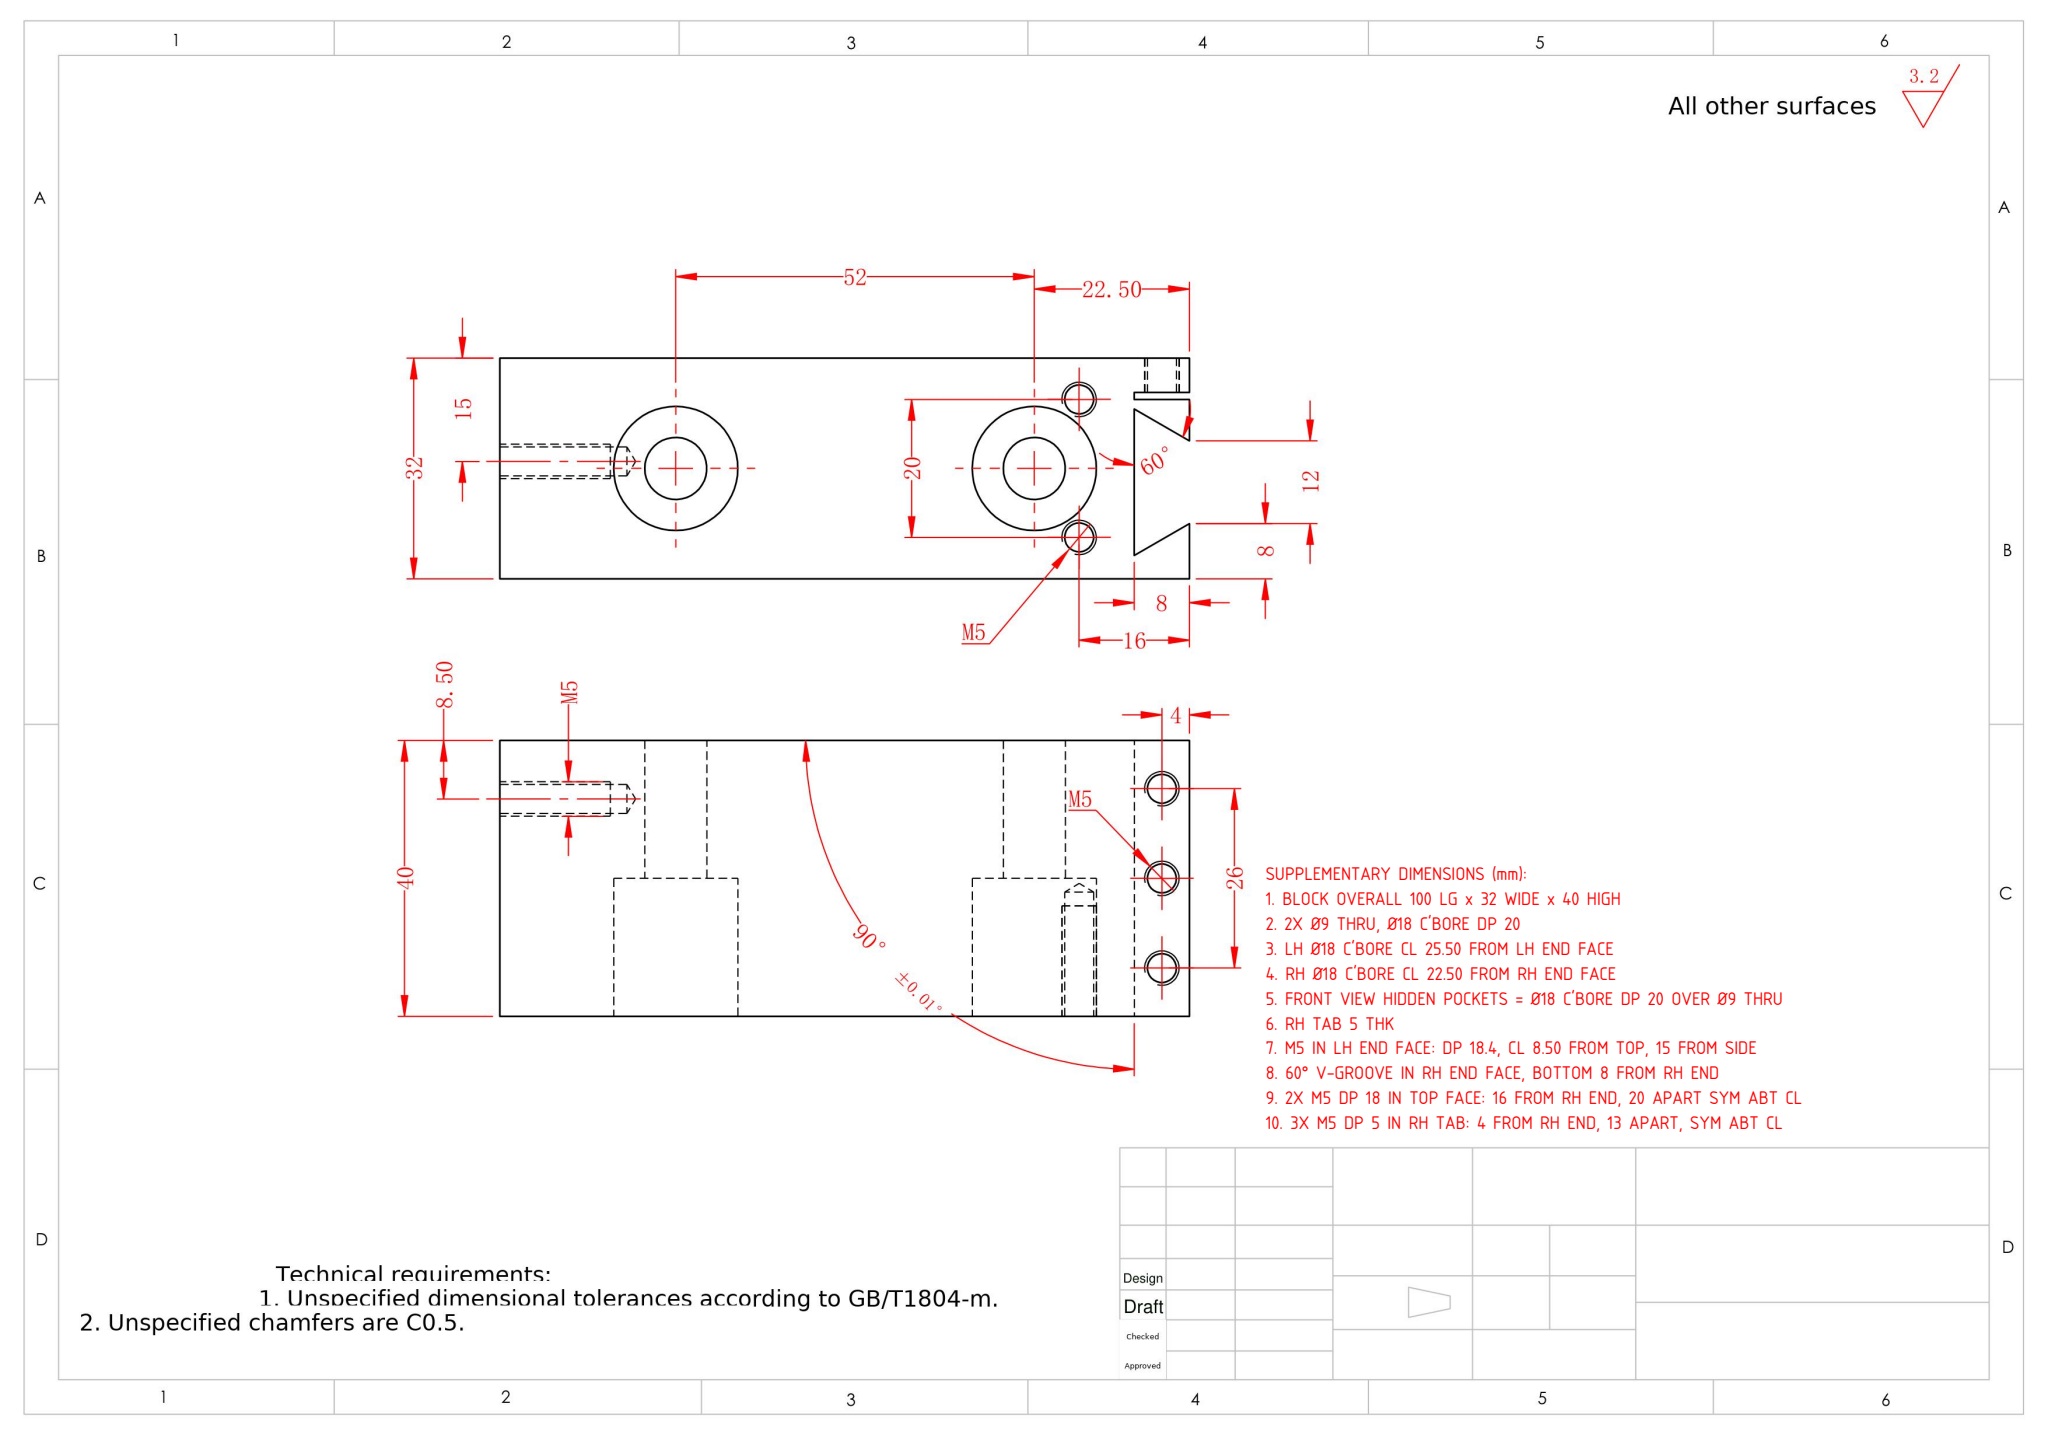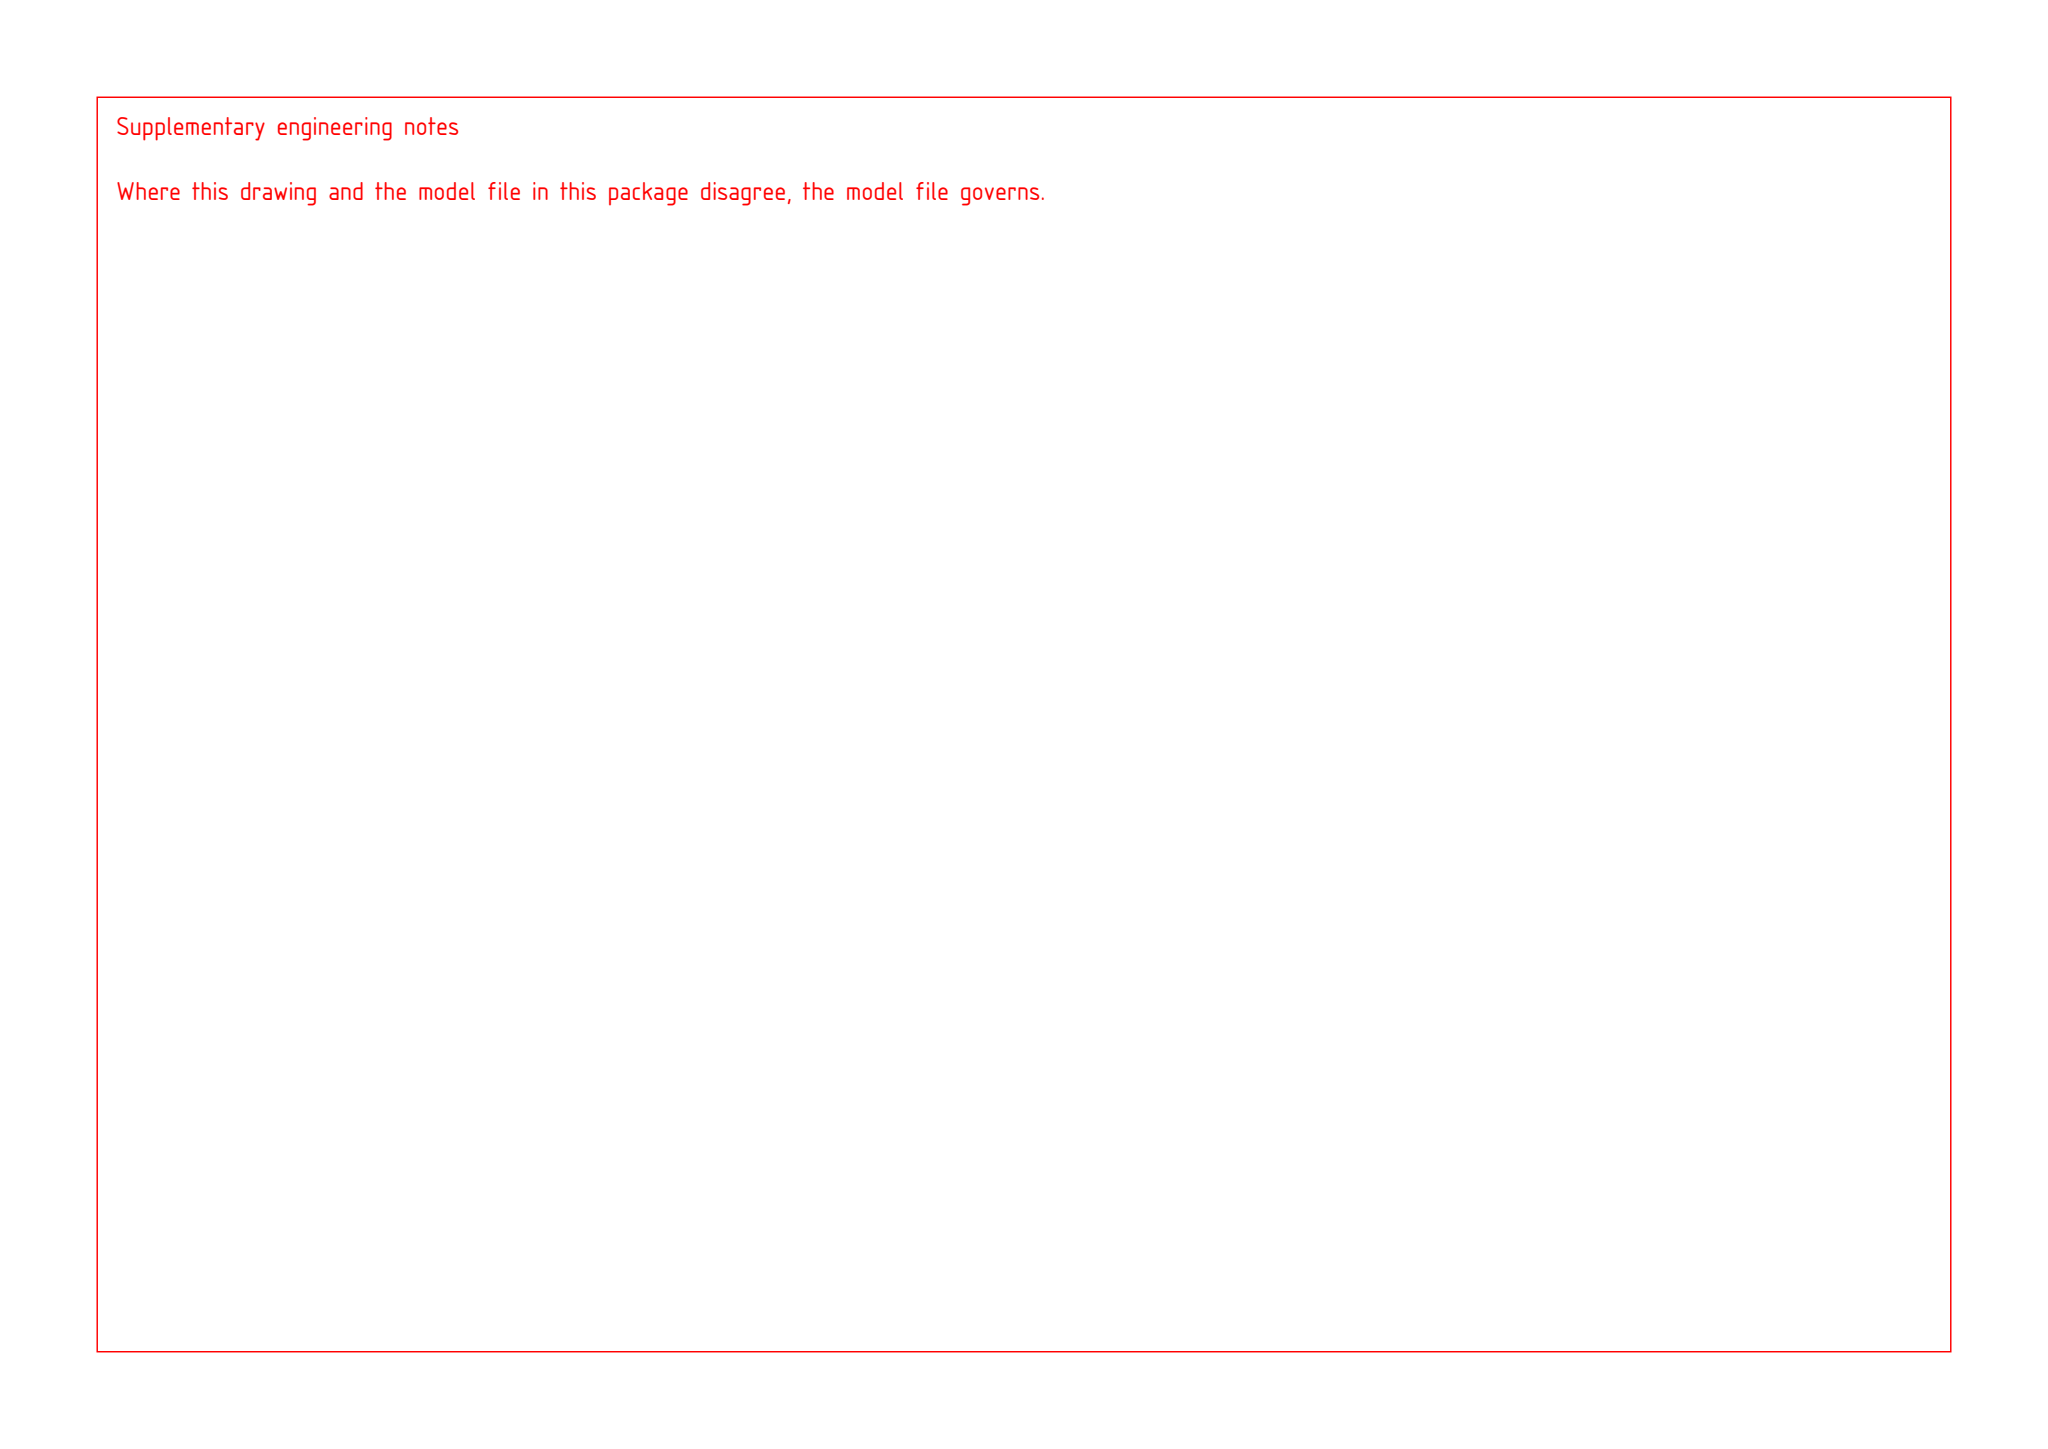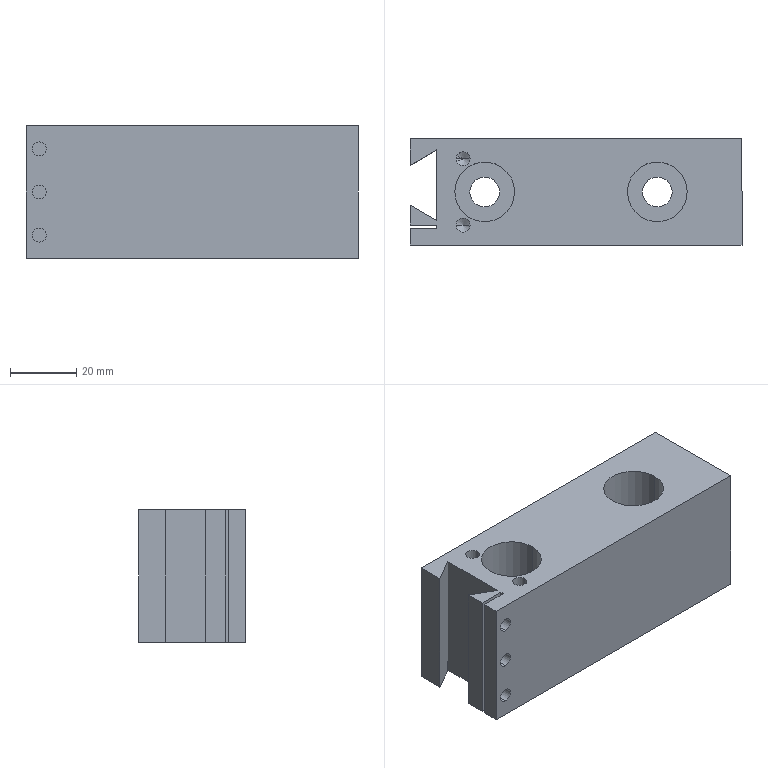Part | SolidWorks | mm | 1 solid | 42 faces | box 100 x 32 x 40 mm | volume 108660 mm3 | cylinder 20 | plane 16 | cone 6 | commonest cylinder face diameters 4.2 x12 18 x4 9 x4
build123d program:
from build123d import *

# Parameters (mm, degrees)
BOSS_EXTRUDE1_DEPTH                                 = 40
CYLINDRICAL_COUNTERSUNK_HOLE_FOR_M8_HEX_D           = 9
CYLINDRICAL_COUNTERSUNK_HOLE_FOR_M8_HEX_CBORE_D     = 18
CYLINDRICAL_COUNTERSUNK_HOLE_FOR_M8_HEX_CBORE_DEPTH = 20
M5_TAPPED_HOLE1_D                                   = 4.2
M5_TAPPED_HOLE1_DEPTH                               = 18
M5_TAPPED_HOLE1_TIP                                 = 1.262
M5_TAPPED_HOLE2_D                                   = 4.2
M5_TAPPED_HOLE2_DEPTH                               = 18.4
M5_TAPPED_HOLE2_TIP                                 = 1.262
M5_TAPPED_HOLE3_D                                   = 4.2
M5_TAPPED_HOLE3_DEPTH                               = 5


with BuildPart() as part:
    # Sketch1 → Boss-Extrude1 (new body)
    with BuildSketch(Plane.XY):
        Polygon((-50, 8), (-42, 12.619), (-42, -8.619), (-50, -4), (-50, -10), (-42, -10), (-42, -11), (-50, -11), (-50, -16), (50, -16), (50, 16), (-50, 16), align=None)
    extrude(amount=BOSS_EXTRUDE1_DEPTH)

    # Cylindrical Countersunk Hole for M8 Hex (through all)
    with Locations(Plane.XY.offset(40)):
        with Locations((-27.5, 0), (24.5, 0)):
            CounterBoreHole(CYLINDRICAL_COUNTERSUNK_HOLE_FOR_M8_HEX_D / 2, CYLINDRICAL_COUNTERSUNK_HOLE_FOR_M8_HEX_CBORE_D / 2, CYLINDRICAL_COUNTERSUNK_HOLE_FOR_M8_HEX_CBORE_DEPTH)

    # M5 Tapped Hole1
    with Locations(Plane.XY.offset(40)):
        with Locations((-34, -10), (-34, 10)):
            Hole(M5_TAPPED_HOLE1_D / 2, depth=M5_TAPPED_HOLE1_DEPTH)
            with Locations((0, 0, -(M5_TAPPED_HOLE1_DEPTH + M5_TAPPED_HOLE1_TIP / 2))):  # 118° drill point
                Cone(0, M5_TAPPED_HOLE1_D / 2, M5_TAPPED_HOLE1_TIP, mode=Mode.SUBTRACT)

    # M5 Tapped Hole2
    with Locations(Plane(origin=(50, 0, 0), x_dir=(0, 0, -1), z_dir=(1, 0, 0))):
        with Locations((-8.5, -1)):
            Hole(M5_TAPPED_HOLE2_D / 2, depth=M5_TAPPED_HOLE2_DEPTH)
            with Locations((0, 0, -(M5_TAPPED_HOLE2_DEPTH + M5_TAPPED_HOLE2_TIP / 2))):  # 118° drill point
                Cone(0, M5_TAPPED_HOLE2_D / 2, M5_TAPPED_HOLE2_TIP, mode=Mode.SUBTRACT)

    # M5 Tapped Hole3
    with Locations(Plane(origin=(0, -16, 0), x_dir=(-1, 0, 0), z_dir=(0, -1, 0))):
        with Locations((46, -33), (46, -20), (46, -7)):
            Hole(M5_TAPPED_HOLE3_D / 2, depth=M5_TAPPED_HOLE3_DEPTH)


solid = part.part